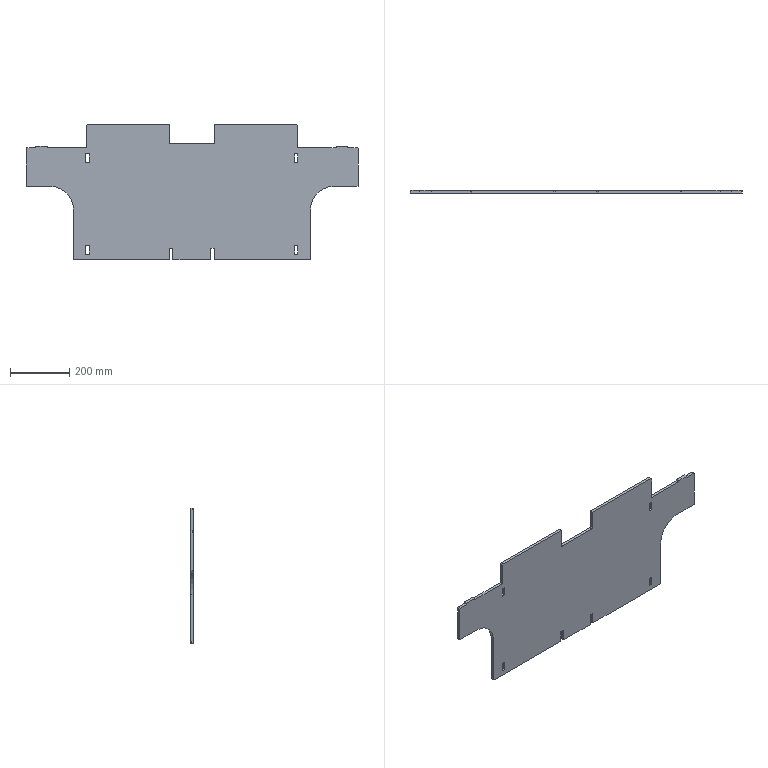Component | SolidWorks | RearUprightPlateConnection-1 | 1 solid | 70 faces | box 1120 x 10 x 458 mm | volume 3914834 mm3 | plane 64 | cylinder 6 | commonest cylinder face diameters 10 x4 160 x2 | material Q235
build123d program:
from build123d import *

# Parameters (mm, degrees)
SKETCH1_2_W             = 10.2
SKETCH1_2_H             = 30
BOSS_EXTRUDE1_DEPTH     = 10
SKETCH2_W               = 12
SKETCH2_H               = 40
CUT_EXTRUDE1_2_DEPTH    = 10
CUT_EXTRUDE1_DEPTH      = 1278.266
CUT_EXTRUDE1_DEPTH_BACK = 1278.266
SKETCH1_W               = 0.6
SKETCH1_H               = 30.6


with BuildPart() as part:
    # Sketch1_2 → Boss-Extrude1 (new body)
    with BuildSketch(Plane.XY):
        with BuildLine():
            Line((424.925, 543.274), (243.425, 543.274))
            Line((243.425, 543.274), (240.425, 540.274))
            Line((240.425, 540.274), (240.425, 493.274))
            Line((240.425, 493.274), (240.425, 463.274))
            Line((240.425, 463.274), (107.867, 463.274))
            Line((107.867, 463.274), (107.867, 468.274))
            Line((107.867, 468.274), (68.867, 468.274))
            Line((68.867, 468.274), (68.867, 463.274))
            Line((68.867, 463.274), (38.925, 463.274))
            Line((38.925, 463.274), (35.925, 460.274))
            Line((35.925, 460.274), (35.925, 383.274))
            Line((35.925, 383.274), (35.925, 333.274))
            Line((35.925, 333.274), (116.425, 333.274))
            ThreePointArc((116.425, 333.274), (172.994, 309.842), (196.425, 253.274))
            Line((196.425, 253.274), (196.425, 96.81))
            Line((196.425, 96.81), (196.425, 91.81))
            Line((196.425, 91.81), (196.425, 90.274))
            ThreePointArc((196.425, 90.274), (197.89, 86.738), (201.425, 85.274))
            Line((201.425, 85.274), (990.425, 85.274))
            ThreePointArc((990.425, 85.274), (993.961, 86.738), (995.425, 90.274))
            Line((995.425, 90.274), (995.425, 91.81))
            Line((995.425, 91.81), (995.425, 96.81))
            Line((995.425, 96.81), (995.425, 253.274))
            ThreePointArc((995.425, 253.274), (1018.857, 309.842), (1075.425, 333.274))
            Line((1075.425, 333.274), (1155.925, 333.274))
            Line((1155.925, 333.274), (1155.925, 383.274))
            Line((1155.925, 383.274), (1155.925, 460.274))
            Line((1155.925, 460.274), (1152.925, 463.274))
            Line((1152.925, 463.274), (1120.925, 463.274))
            Line((1120.925, 463.274), (1120.925, 468.274))
            Line((1120.925, 468.274), (1081.925, 468.274))
            Line((1081.925, 468.274), (1081.925, 463.274))
            Line((1081.925, 463.274), (951.425, 463.274))
            Line((951.425, 463.274), (951.425, 493.274))
            Line((951.425, 493.274), (951.425, 540.274))
            Line((951.425, 540.274), (948.425, 543.274))
            Line((948.425, 543.274), (766.925, 543.274))
            Line((766.925, 543.274), (670.925, 543.274))
            Line((670.925, 543.274), (670.925, 481.274))
            ThreePointArc((670.925, 481.274), (669.461, 477.738), (665.925, 476.274))
            Line((665.925, 476.274), (525.925, 476.274))
            ThreePointArc((525.925, 476.274), (522.39, 477.738), (520.925, 481.274))
            Line((520.925, 481.274), (520.925, 543.274))
            Line((520.925, 543.274), (424.925, 543.274))
        make_face()
        with Locations((243.925, 119.274)):
            Rectangle(SKETCH1_2_W, SKETCH1_2_H, mode=Mode.SUBTRACT)
        with Locations((947.925, 119.274)):
            Rectangle(SKETCH1_2_W, SKETCH1_2_H, mode=Mode.SUBTRACT)
        Polygon((249.025, 413.274), (238.825, 413.274), (238.825, 443.274), (249.025, 443.274), (249.025, 433.274), align=None, mode=Mode.SUBTRACT)
        Polygon((953.025, 443.274), (953.025, 413.274), (942.825, 413.274), (942.825, 433.274), (942.825, 443.274), align=None, mode=Mode.SUBTRACT)
    extrude(amount=BOSS_EXTRUDE1_DEPTH)

    # Sketch2 → Cut-Extrude1_2 (cut)
    with BuildSketch(Plane.XY.offset(10)):
        with Locations((525.229, 105.274)):
            Rectangle(SKETCH2_W, SKETCH2_H)
        with Locations((665.229, 105.274)):
            Rectangle(SKETCH2_W, SKETCH2_H)
    extrude(amount=-CUT_EXTRUDE1_2_DEPTH, mode=Mode.SUBTRACT)

    # Sketch1 → Cut-Extrude1 (cut, two sides: drawn at the far end of the back side and taken through both)
    with BuildSketch(Plane.XY.offset(-CUT_EXTRUDE1_DEPTH_BACK)):
        with Locations((238.579, 119.274)):
            Rectangle(SKETCH1_W, SKETCH1_H)
        with Locations((238.579, 428.274)):
            Rectangle(SKETCH1_W, SKETCH1_H)
    extrude(amount=CUT_EXTRUDE1_DEPTH + CUT_EXTRUDE1_DEPTH_BACK, mode=Mode.SUBTRACT)


solid = part.part

# Placed as in the assembly
solid = solid.moved(Location((-1412.879, -577.326, 2272.431), (90, 0, 0)))